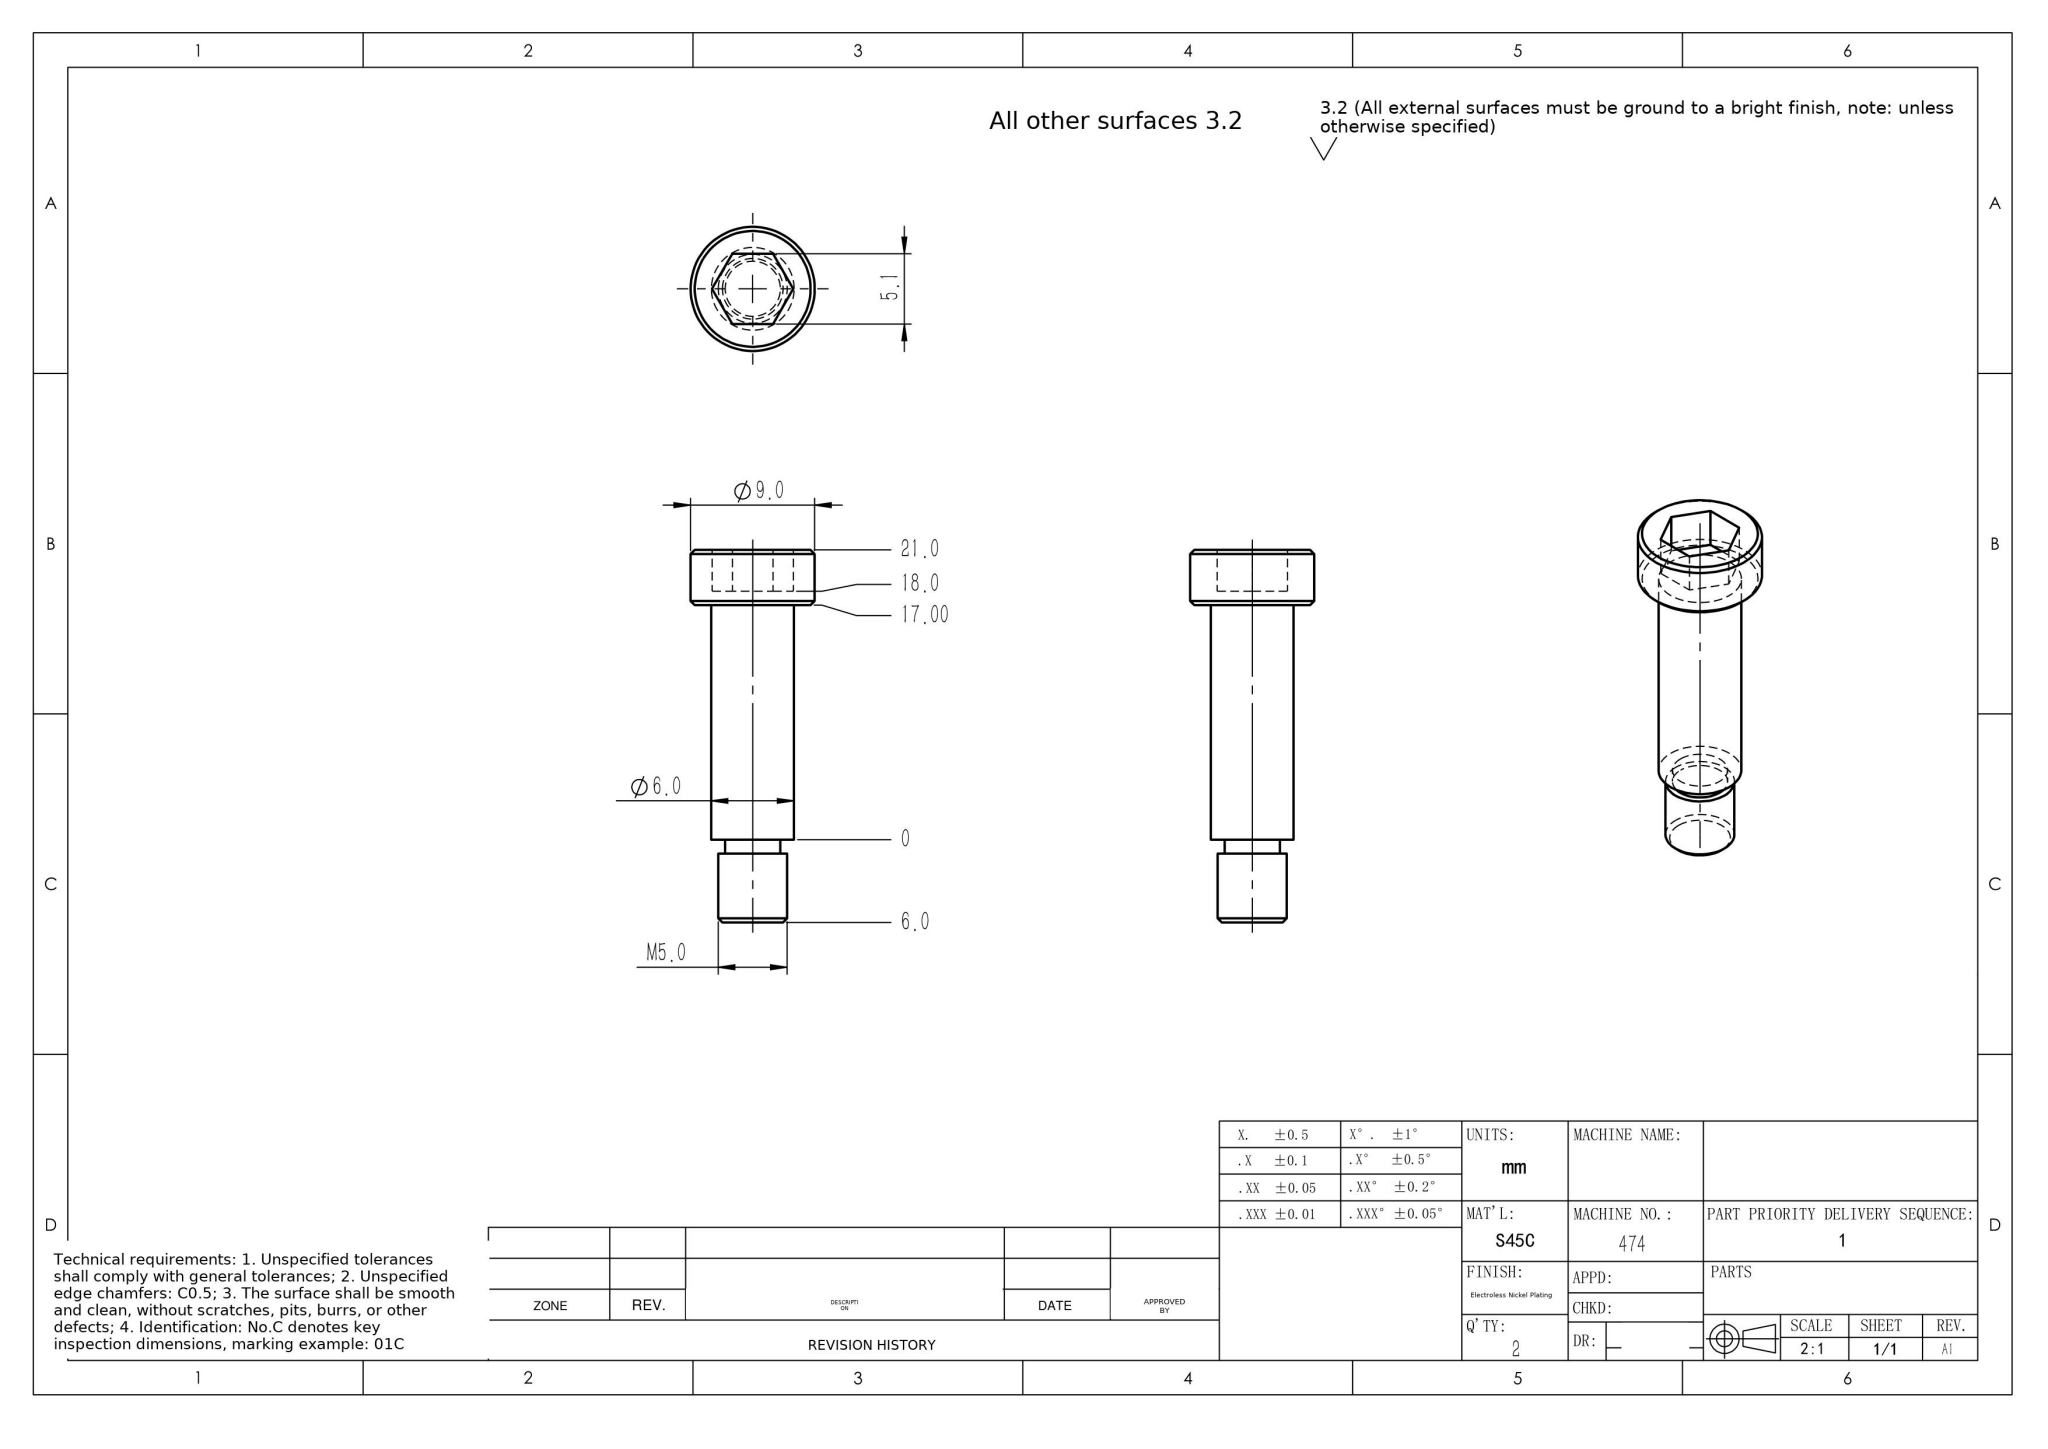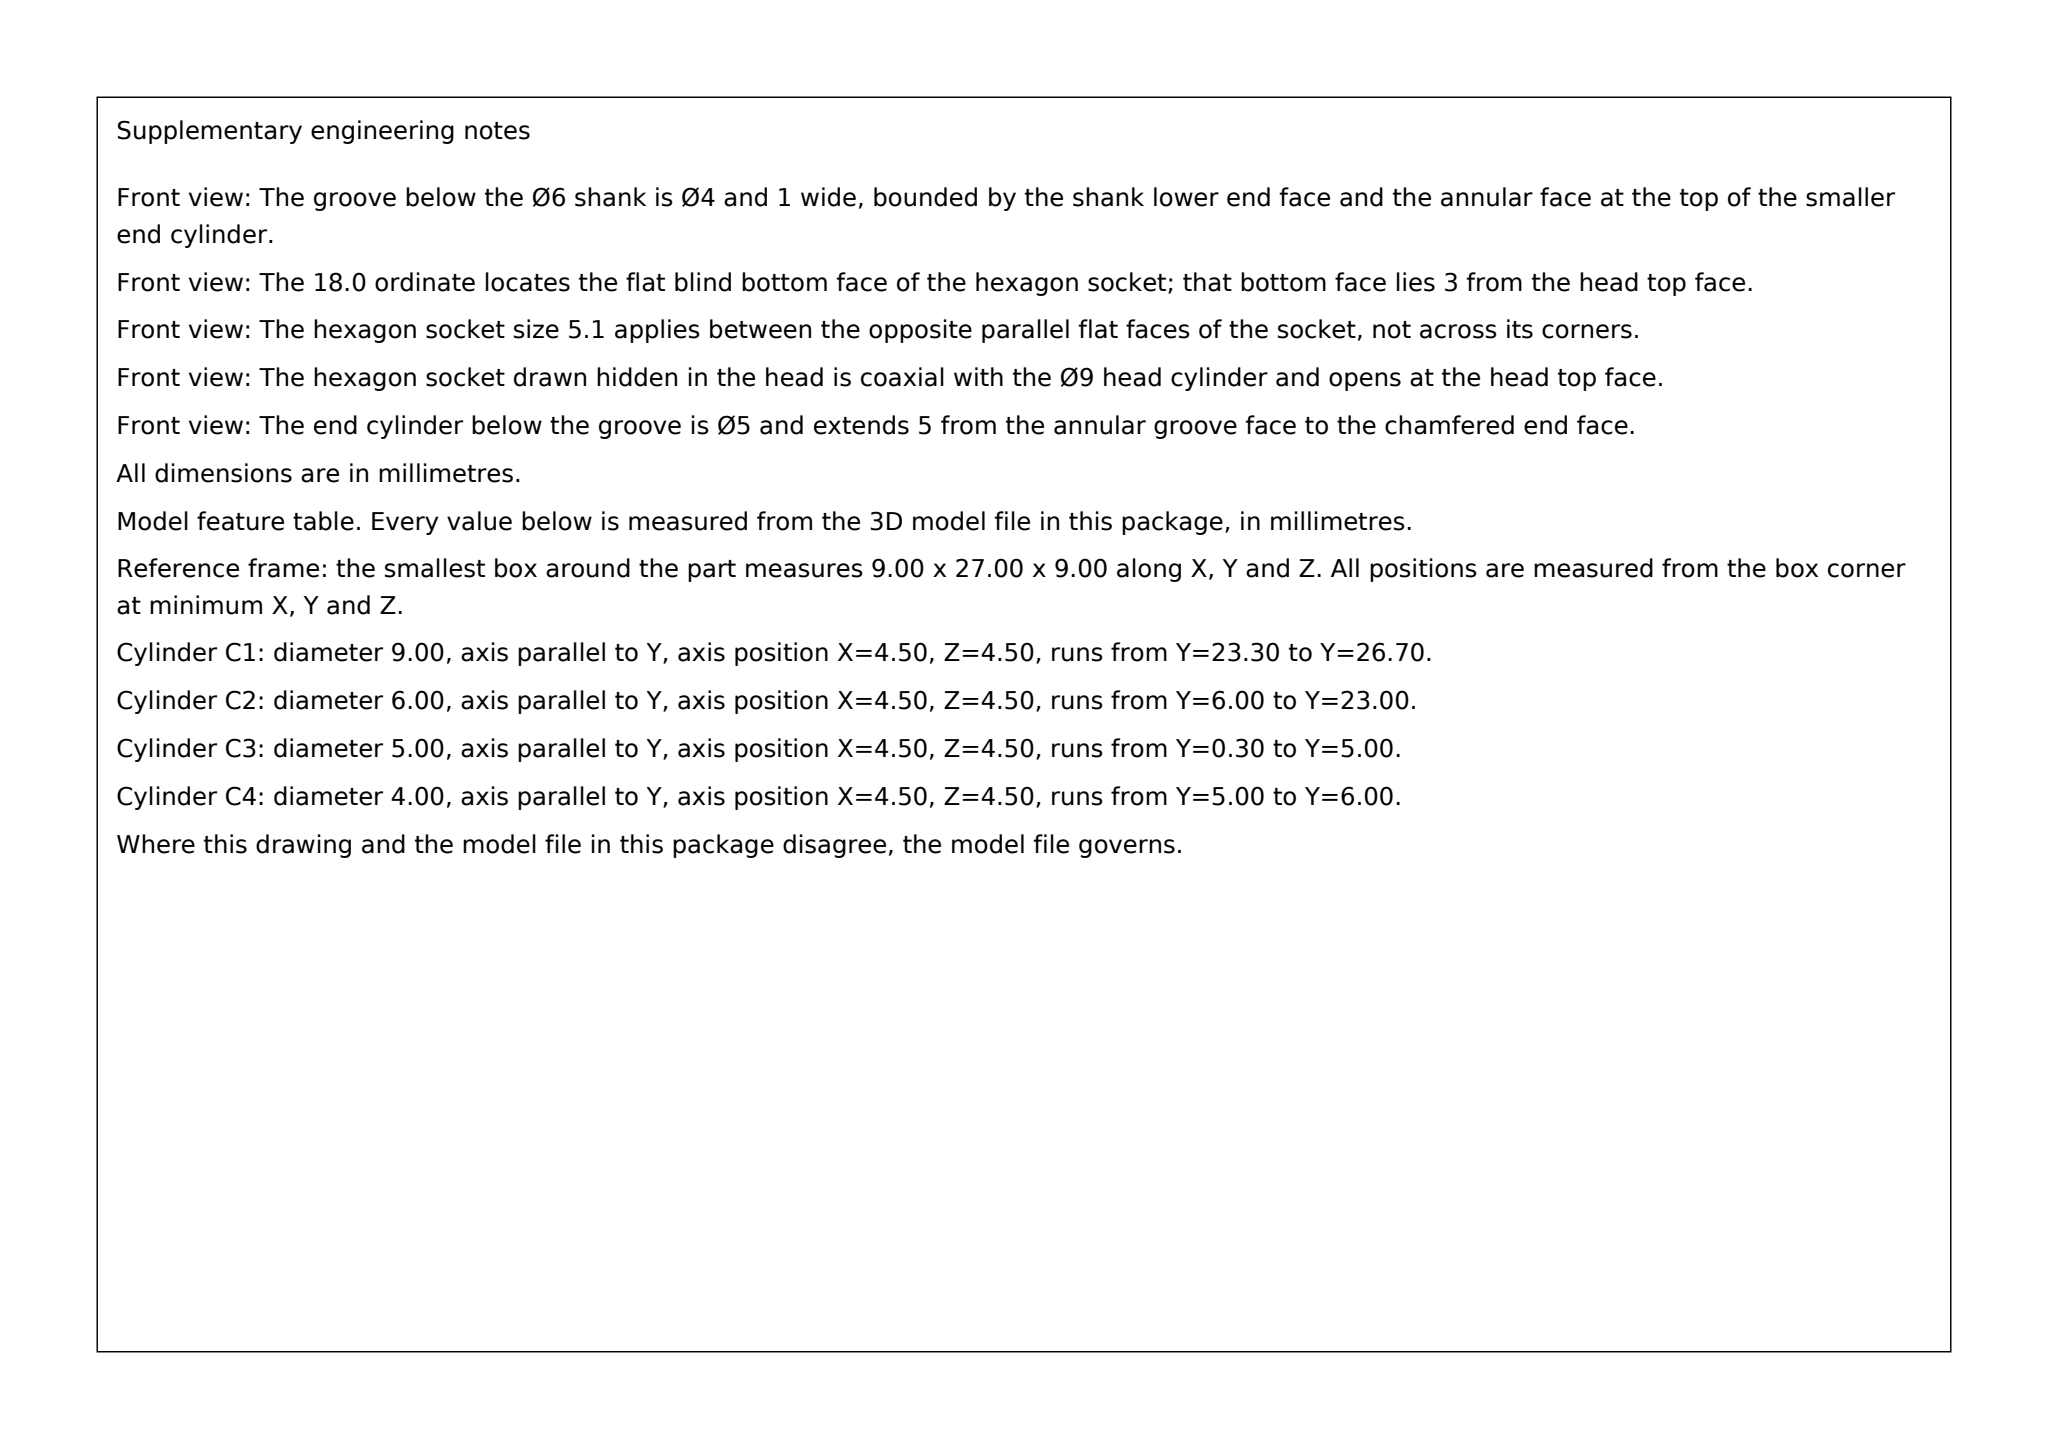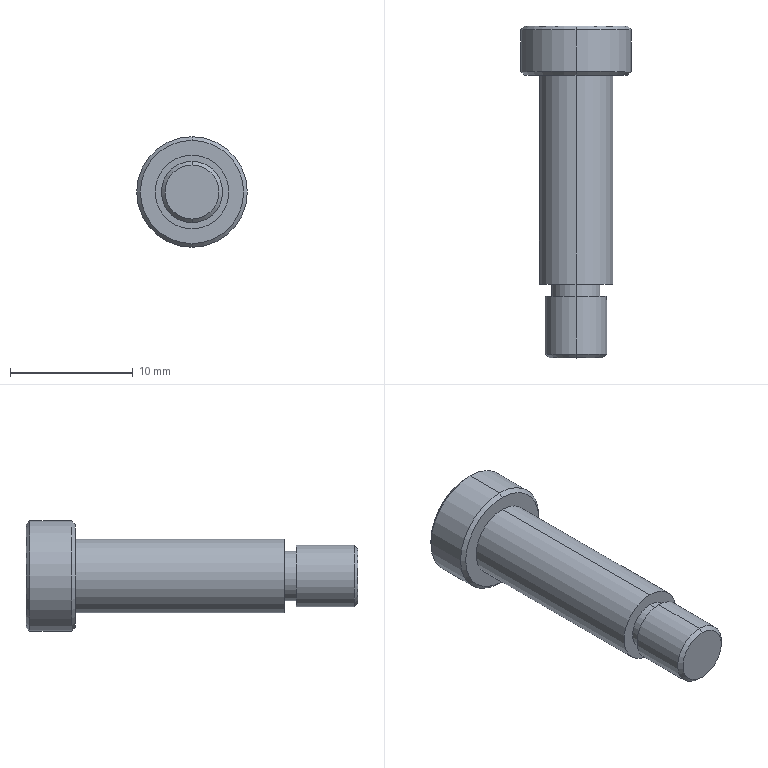Part | SolidWorks | mm | material S45C | 1 solid | 26 faces | box 9 x 27 x 9 mm | volume 775 mm3 | plane 12 | cylinder 8 | cone 6 | commonest cylinder face diameters 5 x2 4 x2 9 x2 6 x2
build123d program:
from build123d import *

# Parameters (mm, degrees)
SKETCH1_R           = 3
BOSS_EXTRUDE1_DEPTH = 17
SKETCH2_R           = 2.5
BOSS_EXTRUDE2_DEPTH = 6
SKETCH3_R           = 4.5
BOSS_EXTRUDE3_DEPTH = 4
CHAMFER1_SIZE       = 0.3
SKETCH4_W           = 1
SKETCH4_H           = 1
CUT_EXTRUDE1_DEPTH  = 3


with BuildPart() as part:
    # Sketch1 → Boss-Extrude1 (new body)
    with BuildSketch(Plane(origin=(0, 0, 0), x_dir=(1, 0, 0), z_dir=(0, 1, 0))):
        with Locations(Location((0, 0, 0), (0, 0, 270))):
            Circle(SKETCH1_R)
    extrude(amount=BOSS_EXTRUDE1_DEPTH)

    # Sketch2 → Boss-Extrude2 (add)
    with BuildSketch(Plane.XZ):
        with Locations(Location((0, 0, 0), (0, 0, 90))):
            Circle(SKETCH2_R)
    extrude(amount=BOSS_EXTRUDE2_DEPTH)

    # Sketch3 → Boss-Extrude3 (add)
    with BuildSketch(Plane(origin=(0, 17, 0), x_dir=(1, 0, 0), z_dir=(0, 1, 0))):
        with Locations(Location((0, 0, 0), (0, 0, 270))):
            Circle(SKETCH3_R)
    extrude(amount=BOSS_EXTRUDE3_DEPTH)

    # Chamfer1
    chamfer1_edges = [part.edges().sort_by_distance(p)[0] for p in [
        (0, -6, -2.5),
        (0, 17, -4.5),
        (0, 21, -4.5),
    ]]
    chamfer(chamfer1_edges, length=CHAMFER1_SIZE)

    # Sketch4 → Cut-Revolve1 (revolve, cut)
    with BuildSketch(Plane.XY, mode=Mode.PRIVATE) as cut_revolve1_sk:
        with Locations((2.5, -0.5)):
            Rectangle(SKETCH4_W, SKETCH4_H)
    revolve(cut_revolve1_sk.sketch.rotate(Axis((0, -5.7, 0), (0, 1, 0)), 90), axis=Axis((0, -5.7, 0), (0, 1, 0)), mode=Mode.SUBTRACT)

    # Sketch5 → Cut-Extrude1 (cut)
    with BuildSketch(Plane(origin=(0, 21, 0), x_dir=(1, 0, 0), z_dir=(0, 1, 0))):
        Polygon((0, 2.944), (-2.55, 1.472), (-2.55, -1.472), (0, -2.944), (2.55, -1.472), (2.55, 1.472), align=None)
    extrude(amount=-CUT_EXTRUDE1_DEPTH, mode=Mode.SUBTRACT)


solid = part.part
STEP:
#1=CARTESIAN_POINT('',(0.,-5.7,2.5));
#2=VERTEX_POINT('',#1);
#3=CARTESIAN_POINT('',(0.,-5.7,-2.5));
#4=VERTEX_POINT('',#3);
#5=CARTESIAN_POINT('',(0.,-5.7,0.));
#6=DIRECTION('',(0.,1.,0.));
#7=DIRECTION('',(0.,0.,-1.));
#8=AXIS2_PLACEMENT_3D('',#5,#6,#7);
#9=CIRCLE('',#8,2.5);
#10=EDGE_CURVE('',#2,#4,#9,.T.);
#11=ORIENTED_EDGE('',*,*,#10,.T.);
#12=CARTESIAN_POINT('',(0.,-1.,-2.5));
#13=VERTEX_POINT('',#12);
#14=CARTESIAN_POINT('',(0.,-6.,-2.5));
#15=DIRECTION('',(0.,1.,0.));
#16=VECTOR('',#15,1000.);
#17=LINE('',#14,#16);
#18=EDGE_CURVE('',#4,#13,#17,.T.);
#19=ORIENTED_EDGE('',*,*,#18,.T.);
#20=CARTESIAN_POINT('',(0.,-1.,2.5));
#21=VERTEX_POINT('',#20);
#22=CARTESIAN_POINT('',(0.,-1.,0.));
#23=DIRECTION('',(0.,-1.,0.));
#24=DIRECTION('',(0.,0.,-1.));
#25=AXIS2_PLACEMENT_3D('',#22,#23,#24);
#26=CIRCLE('',#25,2.5);
#27=EDGE_CURVE('',#13,#21,#26,.T.);
#28=ORIENTED_EDGE('',*,*,#27,.T.);
#29=CARTESIAN_POINT('',(0.,-6.,2.5));
#30=DIRECTION('',(0.,1.,0.));
#31=VECTOR('',#30,1000.);
#32=LINE('',#29,#31);
#33=EDGE_CURVE('',#2,#21,#32,.T.);
#34=ORIENTED_EDGE('',*,*,#33,.F.);
#35=EDGE_LOOP('',(#11,#19,#28,#34));
#36=FACE_OUTER_BOUND('',#35,.T.);
#37=CARTESIAN_POINT('',(0.,-6.,0.));
#38=DIRECTION('',(0.,1.,0.));
#39=DIRECTION('',(0.,0.,1.));
#40=AXIS2_PLACEMENT_3D('',#37,#38,#39);
#41=CYLINDRICAL_SURFACE('',#40,2.5);
#42=ADVANCED_FACE('',(#36),#41,.T.);
#43=CARTESIAN_POINT('',(0.,-6.,-2.2));
#44=VERTEX_POINT('',#43);
#45=CARTESIAN_POINT('',(0.,-6.,2.2));
#46=VERTEX_POINT('',#45);
#47=CARTESIAN_POINT('',(0.,-6.,0.));
#48=DIRECTION('',(0.,-1.,0.));
#49=DIRECTION('',(0.,0.,-1.));
#50=AXIS2_PLACEMENT_3D('',#47,#48,#49);
#51=CIRCLE('',#50,2.2);
#52=EDGE_CURVE('',#44,#46,#51,.T.);
#53=ORIENTED_EDGE('',*,*,#52,.F.);
#54=CARTESIAN_POINT('',(0.,-6.,-2.2));
#55=DIRECTION('',(0.,0.7071,-0.7071));
#56=VECTOR('',#55,1000.);
#57=LINE('',#54,#56);
#58=EDGE_CURVE('',#44,#4,#57,.T.);
#59=ORIENTED_EDGE('',*,*,#58,.T.);
#60=ORIENTED_EDGE('',*,*,#10,.F.);
#61=CARTESIAN_POINT('',(0.,-6.,2.2));
#62=DIRECTION('',(0.,0.7071,0.7071));
#63=VECTOR('',#62,1000.);
#64=LINE('',#61,#63);
#65=EDGE_CURVE('',#46,#2,#64,.T.);
#66=ORIENTED_EDGE('',*,*,#65,.F.);
#67=EDGE_LOOP('',(#53,#59,#60,#66));
#68=FACE_OUTER_BOUND('',#67,.T.);
#69=CARTESIAN_POINT('',(0.,-6.,0.));
#70=DIRECTION('',(0.,1.,0.));
#71=DIRECTION('',(0.,0.,1.));
#72=AXIS2_PLACEMENT_3D('',#69,#70,#71);
#73=CONICAL_SURFACE('',#72,2.2,0.7854);
#74=ADVANCED_FACE('',(#68),#73,.T.);
#75=CARTESIAN_POINT('',(0.,0.,-2.));
#76=VERTEX_POINT('',#75);
#77=CARTESIAN_POINT('',(0.,0.,2.));
#78=VERTEX_POINT('',#77);
#79=CARTESIAN_POINT('',(0.,0.,0.));
#80=DIRECTION('',(0.,-1.,0.));
#81=DIRECTION('',(0.,0.,-1.));
#82=AXIS2_PLACEMENT_3D('',#79,#80,#81);
#83=CIRCLE('',#82,2.);
#84=EDGE_CURVE('',#76,#78,#83,.T.);
#85=ORIENTED_EDGE('',*,*,#84,.T.);
#86=CARTESIAN_POINT('',(0.,-1.,2.));
#87=VERTEX_POINT('',#86);
#88=CARTESIAN_POINT('',(0.,-5.7,2.));
#89=DIRECTION('',(0.,-1.,0.));
#90=VECTOR('',#89,1000.);
#91=LINE('',#88,#90);
#92=EDGE_CURVE('',#78,#87,#91,.T.);
#93=ORIENTED_EDGE('',*,*,#92,.T.);
#94=CARTESIAN_POINT('',(0.,-1.,-2.));
#95=VERTEX_POINT('',#94);
#96=CARTESIAN_POINT('',(0.,-1.,0.));
#97=DIRECTION('',(0.,-1.,0.));
#98=DIRECTION('',(0.,0.,-1.));
#99=AXIS2_PLACEMENT_3D('',#96,#97,#98);
#100=CIRCLE('',#99,2.);
#101=EDGE_CURVE('',#95,#87,#100,.T.);
#102=ORIENTED_EDGE('',*,*,#101,.F.);
#103=CARTESIAN_POINT('',(0.,-5.7,-2.));
#104=DIRECTION('',(0.,-1.,0.));
#105=VECTOR('',#104,1000.);
#106=LINE('',#103,#105);
#107=EDGE_CURVE('',#76,#95,#106,.T.);
#108=ORIENTED_EDGE('',*,*,#107,.F.);
#109=EDGE_LOOP('',(#85,#93,#102,#108));
#110=FACE_OUTER_BOUND('',#109,.T.);
#111=CARTESIAN_POINT('',(0.,-5.7,0.));
#112=DIRECTION('',(0.,-1.,0.));
#113=DIRECTION('',(0.,0.,-1.));
#114=AXIS2_PLACEMENT_3D('',#111,#112,#113);
#115=CYLINDRICAL_SURFACE('',#114,2.);
#116=ADVANCED_FACE('',(#110),#115,.T.);
#117=CARTESIAN_POINT('',(0.,17.,-4.2));
#118=VERTEX_POINT('',#117);
#119=CARTESIAN_POINT('',(0.,17.,4.2));
#120=VERTEX_POINT('',#119);
#121=CARTESIAN_POINT('',(0.,17.,0.));
#122=DIRECTION('',(0.,-1.,0.));
#123=DIRECTION('',(0.,0.,1.));
#124=AXIS2_PLACEMENT_3D('',#121,#122,#123);
#125=CIRCLE('',#124,4.2);
#126=EDGE_CURVE('',#118,#120,#125,.T.);
#127=ORIENTED_EDGE('',*,*,#126,.F.);
#128=CARTESIAN_POINT('',(0.,17.3,-4.5));
#129=VERTEX_POINT('',#128);
#130=CARTESIAN_POINT('',(0.,17.3,-4.5));
#131=DIRECTION('',(0.,0.7071,-0.7071));
#132=VECTOR('',#131,1000.);
#133=LINE('',#130,#132);
#134=EDGE_CURVE('',#118,#129,#133,.T.);
#135=ORIENTED_EDGE('',*,*,#134,.T.);
#136=CARTESIAN_POINT('',(0.,17.3,4.5));
#137=VERTEX_POINT('',#136);
#138=CARTESIAN_POINT('',(0.,17.3,0.));
#139=DIRECTION('',(0.,1.,0.));
#140=DIRECTION('',(0.,0.,1.));
#141=AXIS2_PLACEMENT_3D('',#138,#139,#140);
#142=CIRCLE('',#141,4.5);
#143=EDGE_CURVE('',#137,#129,#142,.T.);
#144=ORIENTED_EDGE('',*,*,#143,.F.);
#145=CARTESIAN_POINT('',(0.,17.3,4.5));
#146=DIRECTION('',(0.,0.7071,0.7071));
#147=VECTOR('',#146,1000.);
#148=LINE('',#145,#147);
#149=EDGE_CURVE('',#120,#137,#148,.T.);
#150=ORIENTED_EDGE('',*,*,#149,.F.);
#151=EDGE_LOOP('',(#127,#135,#144,#150));
#152=FACE_OUTER_BOUND('',#151,.T.);
#153=CARTESIAN_POINT('',(0.,17.3,0.));
#154=DIRECTION('',(0.,1.,0.));
#155=DIRECTION('',(0.,0.,1.));
#156=AXIS2_PLACEMENT_3D('',#153,#154,#155);
#157=CONICAL_SURFACE('',#156,4.5,0.7854);
#158=ADVANCED_FACE('',(#152),#157,.T.);
#159=CARTESIAN_POINT('',(0.,21.,4.2));
#160=VERTEX_POINT('',#159);
#161=CARTESIAN_POINT('',(0.,21.,-4.2));
#162=VERTEX_POINT('',#161);
#163=CARTESIAN_POINT('',(0.,21.,0.));
#164=DIRECTION('',(0.,1.,0.));
#165=DIRECTION('',(0.,0.,1.));
#166=AXIS2_PLACEMENT_3D('',#163,#164,#165);
#167=CIRCLE('',#166,4.2);
#168=EDGE_CURVE('',#160,#162,#167,.T.);
#169=ORIENTED_EDGE('',*,*,#168,.F.);
#170=CARTESIAN_POINT('',(0.,20.7,4.5));
#171=VERTEX_POINT('',#170);
#172=CARTESIAN_POINT('',(0.,21.,4.2));
#173=DIRECTION('',(0.,-0.7071,0.7071));
#174=VECTOR('',#173,1000.);
#175=LINE('',#172,#174);
#176=EDGE_CURVE('',#160,#171,#175,.T.);
#177=ORIENTED_EDGE('',*,*,#176,.T.);
#178=CARTESIAN_POINT('',(0.,20.7,-4.5));
#179=VERTEX_POINT('',#178);
#180=CARTESIAN_POINT('',(0.,20.7,0.));
#181=DIRECTION('',(0.,-1.,0.));
#182=DIRECTION('',(0.,0.,1.));
#183=AXIS2_PLACEMENT_3D('',#180,#181,#182);
#184=CIRCLE('',#183,4.5);
#185=EDGE_CURVE('',#179,#171,#184,.T.);
#186=ORIENTED_EDGE('',*,*,#185,.F.);
#187=CARTESIAN_POINT('',(0.,21.,-4.2));
#188=DIRECTION('',(0.,-0.7071,-0.7071));
#189=VECTOR('',#188,1000.);
#190=LINE('',#187,#189);
#191=EDGE_CURVE('',#162,#179,#190,.T.);
#192=ORIENTED_EDGE('',*,*,#191,.F.);
#193=EDGE_LOOP('',(#169,#177,#186,#192));
#194=FACE_OUTER_BOUND('',#193,.T.);
#195=CARTESIAN_POINT('',(0.,21.,0.));
#196=DIRECTION('',(0.,-1.,0.));
#197=DIRECTION('',(0.,0.,-1.));
#198=AXIS2_PLACEMENT_3D('',#195,#196,#197);
#199=CONICAL_SURFACE('',#198,4.2,0.7854);
#200=ADVANCED_FACE('',(#194),#199,.T.);
#201=ORIENTED_EDGE('',*,*,#185,.T.);
#202=CARTESIAN_POINT('',(0.,21.,4.5));
#203=DIRECTION('',(0.,-1.,0.));
#204=VECTOR('',#203,1000.);
#205=LINE('',#202,#204);
#206=EDGE_CURVE('',#171,#137,#205,.T.);
#207=ORIENTED_EDGE('',*,*,#206,.T.);
#208=ORIENTED_EDGE('',*,*,#143,.T.);
#209=CARTESIAN_POINT('',(0.,21.,-4.5));
#210=DIRECTION('',(0.,-1.,0.));
#211=VECTOR('',#210,1000.);
#212=LINE('',#209,#211);
#213=EDGE_CURVE('',#179,#129,#212,.T.);
#214=ORIENTED_EDGE('',*,*,#213,.F.);
#215=EDGE_LOOP('',(#201,#207,#208,#214));
#216=FACE_OUTER_BOUND('',#215,.T.);
#217=CARTESIAN_POINT('',(0.,21.,0.));
#218=DIRECTION('',(0.,-1.,0.));
#219=DIRECTION('',(0.,0.,-1.));
#220=AXIS2_PLACEMENT_3D('',#217,#218,#219);
#221=CYLINDRICAL_SURFACE('',#220,4.5);
#222=ADVANCED_FACE('',(#216),#221,.T.);
#223=CARTESIAN_POINT('',(0.,17.,3.));
#224=VERTEX_POINT('',#223);
#225=CARTESIAN_POINT('',(0.,17.,-3.));
#226=VERTEX_POINT('',#225);
#227=CARTESIAN_POINT('',(0.,17.,0.));
#228=DIRECTION('',(0.,1.,0.));
#229=DIRECTION('',(0.,0.,1.));
#230=AXIS2_PLACEMENT_3D('',#227,#228,#229);
#231=CIRCLE('',#230,3.);
#232=EDGE_CURVE('',#224,#226,#231,.T.);
#233=ORIENTED_EDGE('',*,*,#232,.F.);
#234=CARTESIAN_POINT('',(0.,0.,3.));
#235=VERTEX_POINT('',#234);
#236=CARTESIAN_POINT('',(0.,17.,3.));
#237=DIRECTION('',(0.,-1.,0.));
#238=VECTOR('',#237,1000.);
#239=LINE('',#236,#238);
#240=EDGE_CURVE('',#224,#235,#239,.T.);
#241=ORIENTED_EDGE('',*,*,#240,.T.);
#242=CARTESIAN_POINT('',(0.,0.,-3.));
#243=VERTEX_POINT('',#242);
#244=CARTESIAN_POINT('',(0.,0.,0.));
#245=DIRECTION('',(0.,1.,0.));
#246=DIRECTION('',(0.,0.,1.));
#247=AXIS2_PLACEMENT_3D('',#244,#245,#246);
#248=CIRCLE('',#247,3.);
#249=EDGE_CURVE('',#235,#243,#248,.T.);
#250=ORIENTED_EDGE('',*,*,#249,.T.);
#251=CARTESIAN_POINT('',(0.,17.,-3.));
#252=DIRECTION('',(0.,-1.,0.));
#253=VECTOR('',#252,1000.);
#254=LINE('',#251,#253);
#255=EDGE_CURVE('',#226,#243,#254,.T.);
#256=ORIENTED_EDGE('',*,*,#255,.F.);
#257=EDGE_LOOP('',(#233,#241,#250,#256));
#258=FACE_OUTER_BOUND('',#257,.T.);
#259=CARTESIAN_POINT('',(0.,17.,0.));
#260=DIRECTION('',(0.,-1.,0.));
#261=DIRECTION('',(0.,0.,-1.));
#262=AXIS2_PLACEMENT_3D('',#259,#260,#261);
#263=CYLINDRICAL_SURFACE('',#262,3.);
#264=ADVANCED_FACE('',(#258),#263,.T.);
#265=ORIENTED_EDGE('',*,*,#240,.F.);
#266=CARTESIAN_POINT('',(0.,17.,0.));
#267=DIRECTION('',(0.,1.,0.));
#268=DIRECTION('',(0.,0.,1.));
#269=AXIS2_PLACEMENT_3D('',#266,#267,#268);
#270=CIRCLE('',#269,3.);
#271=EDGE_CURVE('',#226,#224,#270,.T.);
#272=ORIENTED_EDGE('',*,*,#271,.F.);
#273=ORIENTED_EDGE('',*,*,#255,.T.);
#274=CARTESIAN_POINT('',(0.,0.,0.));
#275=DIRECTION('',(0.,1.,0.));
#276=DIRECTION('',(0.,0.,1.));
#277=AXIS2_PLACEMENT_3D('',#274,#275,#276);
#278=CIRCLE('',#277,3.);
#279=EDGE_CURVE('',#243,#235,#278,.T.);
#280=ORIENTED_EDGE('',*,*,#279,.T.);
#281=EDGE_LOOP('',(#265,#272,#273,#280));
#282=FACE_OUTER_BOUND('',#281,.T.);
#283=CARTESIAN_POINT('',(0.,17.,0.));
#284=DIRECTION('',(0.,-1.,0.));
#285=DIRECTION('',(0.,0.,-1.));
#286=AXIS2_PLACEMENT_3D('',#283,#284,#285);
#287=CYLINDRICAL_SURFACE('',#286,3.);
#288=ADVANCED_FACE('',(#282),#287,.T.);
#289=ORIENTED_EDGE('',*,*,#279,.F.);
#290=ORIENTED_EDGE('',*,*,#249,.F.);
#291=EDGE_LOOP('',(#289,#290));
#292=FACE_OUTER_BOUND('',#291,.T.);
#293=ORIENTED_EDGE('',*,*,#84,.F.);
#294=CARTESIAN_POINT('',(0.,0.,0.));
#295=DIRECTION('',(0.,-1.,0.));
#296=DIRECTION('',(0.,0.,-1.));
#297=AXIS2_PLACEMENT_3D('',#294,#295,#296);
#298=CIRCLE('',#297,2.);
#299=EDGE_CURVE('',#78,#76,#298,.T.);
#300=ORIENTED_EDGE('',*,*,#299,.F.);
#301=EDGE_LOOP('',(#293,#300));
#302=FACE_BOUND('',#301,.T.);
#303=CARTESIAN_POINT('',(0.,0.,0.));
#304=DIRECTION('',(0.,1.,0.));
#305=DIRECTION('',(0.,0.,1.));
#306=AXIS2_PLACEMENT_3D('',#303,#304,#305);
#307=PLANE('',#306);
#308=ADVANCED_FACE('',(#292,#302),#307,.F.);
#309=ORIENTED_EDGE('',*,*,#206,.F.);
#310=CARTESIAN_POINT('',(0.,20.7,0.));
#311=DIRECTION('',(0.,-1.,0.));
#312=DIRECTION('',(0.,0.,1.));
#313=AXIS2_PLACEMENT_3D('',#310,#311,#312);
#314=CIRCLE('',#313,4.5);
#315=EDGE_CURVE('',#171,#179,#314,.T.);
#316=ORIENTED_EDGE('',*,*,#315,.T.);
#317=ORIENTED_EDGE('',*,*,#213,.T.);
#318=CARTESIAN_POINT('',(0.,17.3,0.));
#319=DIRECTION('',(0.,1.,0.));
#320=DIRECTION('',(0.,0.,1.));
#321=AXIS2_PLACEMENT_3D('',#318,#319,#320);
#322=CIRCLE('',#321,4.5);
#323=EDGE_CURVE('',#129,#137,#322,.T.);
#324=ORIENTED_EDGE('',*,*,#323,.T.);
#325=EDGE_LOOP('',(#309,#316,#317,#324));
#326=FACE_OUTER_BOUND('',#325,.T.);
#327=CARTESIAN_POINT('',(0.,21.,0.));
#328=DIRECTION('',(0.,-1.,0.));
#329=DIRECTION('',(0.,0.,-1.));
#330=AXIS2_PLACEMENT_3D('',#327,#328,#329);
#331=CYLINDRICAL_SURFACE('',#330,4.5);
#332=ADVANCED_FACE('',(#326),#331,.T.);
#333=CARTESIAN_POINT('',(2.55,21.,-1.472));
#334=VERTEX_POINT('',#333);
#335=CARTESIAN_POINT('',(0.,21.,-2.944));
#336=VERTEX_POINT('',#335);
#337=CARTESIAN_POINT('',(2.55,21.,-1.472));
#338=DIRECTION('',(-0.866,0.,-0.5));
#339=VECTOR('',#338,1000.);
#340=LINE('',#337,#339);
#341=EDGE_CURVE('',#334,#336,#340,.T.);
#342=ORIENTED_EDGE('',*,*,#341,.F.);
#343=CARTESIAN_POINT('',(2.55,21.,1.472));
#344=VERTEX_POINT('',#343);
#345=CARTESIAN_POINT('',(2.55,21.,1.472));
#346=DIRECTION('',(0.,0.,-1.));
#347=VECTOR('',#346,1000.);
#348=LINE('',#345,#347);
#349=EDGE_CURVE('',#344,#334,#348,.T.);
#350=ORIENTED_EDGE('',*,*,#349,.F.);
#351=CARTESIAN_POINT('',(0.,21.,2.944));
#352=VERTEX_POINT('',#351);
#353=CARTESIAN_POINT('',(0.,21.,2.944));
#354=DIRECTION('',(0.866,0.,-0.5));
#355=VECTOR('',#354,1000.);
#356=LINE('',#353,#355);
#357=EDGE_CURVE('',#352,#344,#356,.T.);
#358=ORIENTED_EDGE('',*,*,#357,.F.);
#359=CARTESIAN_POINT('',(-2.55,21.,1.472));
#360=VERTEX_POINT('',#359);
#361=CARTESIAN_POINT('',(-2.55,21.,1.472));
#362=DIRECTION('',(0.866,0.,0.5));
#363=VECTOR('',#362,1000.);
#364=LINE('',#361,#363);
#365=EDGE_CURVE('',#360,#352,#364,.T.);
#366=ORIENTED_EDGE('',*,*,#365,.F.);
#367=CARTESIAN_POINT('',(-2.55,21.,-1.472));
#368=VERTEX_POINT('',#367);
#369=CARTESIAN_POINT('',(-2.55,21.,-1.472));
#370=DIRECTION('',(0.,0.,1.));
#371=VECTOR('',#370,1000.);
#372=LINE('',#369,#371);
#373=EDGE_CURVE('',#368,#360,#372,.T.);
#374=ORIENTED_EDGE('',*,*,#373,.F.);
#375=CARTESIAN_POINT('',(0.,21.,-2.944));
#376=DIRECTION('',(-0.866,0.,0.5));
#377=VECTOR('',#376,1000.);
#378=LINE('',#375,#377);
#379=EDGE_CURVE('',#336,#368,#378,.T.);
#380=ORIENTED_EDGE('',*,*,#379,.F.);
#381=EDGE_LOOP('',(#342,#350,#358,#366,#374,#380));
#382=FACE_BOUND('',#381,.T.);
#383=CARTESIAN_POINT('',(0.,21.,0.));
#384=DIRECTION('',(0.,1.,0.));
#385=DIRECTION('',(0.,0.,1.));
#386=AXIS2_PLACEMENT_3D('',#383,#384,#385);
#387=CIRCLE('',#386,4.2);
#388=EDGE_CURVE('',#162,#160,#387,.T.);
#389=ORIENTED_EDGE('',*,*,#388,.T.);
#390=ORIENTED_EDGE('',*,*,#168,.T.);
#391=EDGE_LOOP('',(#389,#390));
#392=FACE_OUTER_BOUND('',#391,.T.);
#393=CARTESIAN_POINT('',(0.,21.,0.));
#394=DIRECTION('',(0.,1.,0.));
#395=DIRECTION('',(0.,0.,1.));
#396=AXIS2_PLACEMENT_3D('',#393,#394,#395);
#397=PLANE('',#396);
#398=ADVANCED_FACE('',(#382,#392),#397,.T.);
#399=CARTESIAN_POINT('',(0.,17.,0.));
#400=DIRECTION('',(0.,-1.,0.));
#401=DIRECTION('',(0.,0.,1.));
#402=AXIS2_PLACEMENT_3D('',#399,#400,#401);
#403=CIRCLE('',#402,4.2);
#404=EDGE_CURVE('',#120,#118,#403,.T.);
#405=ORIENTED_EDGE('',*,*,#404,.T.);
#406=ORIENTED_EDGE('',*,*,#126,.T.);
#407=EDGE_LOOP('',(#405,#406));
#408=FACE_OUTER_BOUND('',#407,.T.);
#409=ORIENTED_EDGE('',*,*,#271,.T.);
#410=ORIENTED_EDGE('',*,*,#232,.T.);
#411=EDGE_LOOP('',(#409,#410));
#412=FACE_BOUND('',#411,.T.);
#413=CARTESIAN_POINT('',(0.,17.,0.));
#414=DIRECTION('',(0.,1.,0.));
#415=DIRECTION('',(0.,0.,1.));
#416=AXIS2_PLACEMENT_3D('',#413,#414,#415);
#417=PLANE('',#416);
#418=ADVANCED_FACE('',(#408,#412),#417,.F.);
#419=ORIENTED_EDGE('',*,*,#176,.F.);
#420=ORIENTED_EDGE('',*,*,#388,.F.);
#421=ORIENTED_EDGE('',*,*,#191,.T.);
#422=ORIENTED_EDGE('',*,*,#315,.F.);
#423=EDGE_LOOP('',(#419,#420,#421,#422));
#424=FACE_OUTER_BOUND('',#423,.T.);
#425=CARTESIAN_POINT('',(0.,21.,0.));
#426=DIRECTION('',(0.,-1.,0.));
#427=DIRECTION('',(0.,0.,-1.));
#428=AXIS2_PLACEMENT_3D('',#425,#426,#427);
#429=CONICAL_SURFACE('',#428,4.2,0.7854);
#430=ADVANCED_FACE('',(#424),#429,.T.);
#431=ORIENTED_EDGE('',*,*,#134,.F.);
#432=ORIENTED_EDGE('',*,*,#404,.F.);
#433=ORIENTED_EDGE('',*,*,#149,.T.);
#434=ORIENTED_EDGE('',*,*,#323,.F.);
#435=EDGE_LOOP('',(#431,#432,#433,#434));
#436=FACE_OUTER_BOUND('',#435,.T.);
#437=CARTESIAN_POINT('',(0.,17.3,0.));
#438=DIRECTION('',(0.,1.,0.));
#439=DIRECTION('',(0.,0.,1.));
#440=AXIS2_PLACEMENT_3D('',#437,#438,#439);
#441=CONICAL_SURFACE('',#440,4.5,0.7854);
#442=ADVANCED_FACE('',(#436),#441,.T.);
#443=ORIENTED_EDGE('',*,*,#101,.T.);
#444=CARTESIAN_POINT('',(0.,-1.,0.));
#445=DIRECTION('',(0.,-1.,0.));
#446=DIRECTION('',(0.,0.,-1.));
#447=AXIS2_PLACEMENT_3D('',#444,#445,#446);
#448=CIRCLE('',#447,2.);
#449=EDGE_CURVE('',#87,#95,#448,.T.);
#450=ORIENTED_EDGE('',*,*,#449,.T.);
#451=EDGE_LOOP('',(#443,#450));
#452=FACE_BOUND('',#451,.T.);
#453=CARTESIAN_POINT('',(0.,-1.,0.));
#454=DIRECTION('',(0.,-1.,0.));
#455=DIRECTION('',(0.,0.,-1.));
#456=AXIS2_PLACEMENT_3D('',#453,#454,#455);
#457=CIRCLE('',#456,2.5);
#458=EDGE_CURVE('',#21,#13,#457,.T.);
#459=ORIENTED_EDGE('',*,*,#458,.F.);
#460=ORIENTED_EDGE('',*,*,#27,.F.);
#461=EDGE_LOOP('',(#459,#460));
#462=FACE_OUTER_BOUND('',#461,.T.);
#463=CARTESIAN_POINT('',(2.,-1.,0.));
#464=DIRECTION('',(0.,-1.,0.));
#465=DIRECTION('',(0.,0.,-1.));
#466=AXIS2_PLACEMENT_3D('',#463,#464,#465);
#467=PLANE('',#466);
#468=ADVANCED_FACE('',(#452,#462),#467,.F.);
#469=ORIENTED_EDGE('',*,*,#92,.F.);
#470=ORIENTED_EDGE('',*,*,#299,.T.);
#471=ORIENTED_EDGE('',*,*,#107,.T.);
#472=ORIENTED_EDGE('',*,*,#449,.F.);
#473=EDGE_LOOP('',(#469,#470,#471,#472));
#474=FACE_OUTER_BOUND('',#473,.T.);
#475=CARTESIAN_POINT('',(0.,-5.7,0.));
#476=DIRECTION('',(0.,-1.,0.));
#477=DIRECTION('',(0.,0.,-1.));
#478=AXIS2_PLACEMENT_3D('',#475,#476,#477);
#479=CYLINDRICAL_SURFACE('',#478,2.);
#480=ADVANCED_FACE('',(#474),#479,.T.);
#481=CARTESIAN_POINT('',(0.,-6.,0.));
#482=DIRECTION('',(0.,-1.,0.));
#483=DIRECTION('',(0.,0.,-1.));
#484=AXIS2_PLACEMENT_3D('',#481,#482,#483);
#485=CIRCLE('',#484,2.2);
#486=EDGE_CURVE('',#46,#44,#485,.T.);
#487=ORIENTED_EDGE('',*,*,#486,.T.);
#488=ORIENTED_EDGE('',*,*,#52,.T.);
#489=EDGE_LOOP('',(#487,#488));
#490=FACE_OUTER_BOUND('',#489,.T.);
#491=CARTESIAN_POINT('',(0.,-6.,0.));
#492=DIRECTION('',(0.,-1.,0.));
#493=DIRECTION('',(0.,0.,-1.));
#494=AXIS2_PLACEMENT_3D('',#491,#492,#493);
#495=PLANE('',#494);
#496=ADVANCED_FACE('',(#490),#495,.T.);
#497=ORIENTED_EDGE('',*,*,#58,.F.);
#498=ORIENTED_EDGE('',*,*,#486,.F.);
#499=ORIENTED_EDGE('',*,*,#65,.T.);
#500=CARTESIAN_POINT('',(0.,-5.7,0.));
#501=DIRECTION('',(0.,1.,0.));
#502=DIRECTION('',(0.,0.,-1.));
#503=AXIS2_PLACEMENT_3D('',#500,#501,#502);
#504=CIRCLE('',#503,2.5);
#505=EDGE_CURVE('',#4,#2,#504,.T.);
#506=ORIENTED_EDGE('',*,*,#505,.F.);
#507=EDGE_LOOP('',(#497,#498,#499,#506));
#508=FACE_OUTER_BOUND('',#507,.T.);
#509=CARTESIAN_POINT('',(0.,-6.,0.));
#510=DIRECTION('',(0.,1.,0.));
#511=DIRECTION('',(0.,0.,1.));
#512=AXIS2_PLACEMENT_3D('',#509,#510,#511);
#513=CONICAL_SURFACE('',#512,2.2,0.7854);
#514=ADVANCED_FACE('',(#508),#513,.T.);
#515=ORIENTED_EDGE('',*,*,#18,.F.);
#516=ORIENTED_EDGE('',*,*,#505,.T.);
#517=ORIENTED_EDGE('',*,*,#33,.T.);
#518=ORIENTED_EDGE('',*,*,#458,.T.);
#519=EDGE_LOOP('',(#515,#516,#517,#518));
#520=FACE_OUTER_BOUND('',#519,.T.);
#521=CARTESIAN_POINT('',(0.,-6.,0.));
#522=DIRECTION('',(0.,1.,0.));
#523=DIRECTION('',(0.,0.,1.));
#524=AXIS2_PLACEMENT_3D('',#521,#522,#523);
#525=CYLINDRICAL_SURFACE('',#524,2.5);
#526=ADVANCED_FACE('',(#520),#525,.T.);
#527=ORIENTED_EDGE('',*,*,#341,.T.);
#528=CARTESIAN_POINT('',(0.,18.,-2.944));
#529=VERTEX_POINT('',#528);
#530=CARTESIAN_POINT('',(0.,18.,-2.944));
#531=DIRECTION('',(0.,1.,0.));
#532=VECTOR('',#531,1000.);
#533=LINE('',#530,#532);
#534=EDGE_CURVE('',#529,#336,#533,.T.);
#535=ORIENTED_EDGE('',*,*,#534,.F.);
#536=CARTESIAN_POINT('',(2.55,18.,-1.472));
#537=VERTEX_POINT('',#536);
#538=CARTESIAN_POINT('',(2.55,18.,-1.472));
#539=DIRECTION('',(-0.866,0.,-0.5));
#540=VECTOR('',#539,1000.);
#541=LINE('',#538,#540);
#542=EDGE_CURVE('',#537,#529,#541,.T.);
#543=ORIENTED_EDGE('',*,*,#542,.F.);
#544=CARTESIAN_POINT('',(2.55,18.,-1.472));
#545=DIRECTION('',(0.,1.,0.));
#546=VECTOR('',#545,1000.);
#547=LINE('',#544,#546);
#548=EDGE_CURVE('',#537,#334,#547,.T.);
#549=ORIENTED_EDGE('',*,*,#548,.T.);
#550=EDGE_LOOP('',(#527,#535,#543,#549));
#551=FACE_OUTER_BOUND('',#550,.T.);
#552=CARTESIAN_POINT('',(2.55,18.,-1.472));
#553=DIRECTION('',(0.5,0.,-0.866));
#554=DIRECTION('',(-0.866,0.,-0.5));
#555=AXIS2_PLACEMENT_3D('',#552,#553,#554);
#556=PLANE('',#555);
#557=ADVANCED_FACE('',(#551),#556,.F.);
#558=ORIENTED_EDGE('',*,*,#349,.T.);
#559=ORIENTED_EDGE('',*,*,#548,.F.);
#560=CARTESIAN_POINT('',(2.55,18.,1.472));
#561=VERTEX_POINT('',#560);
#562=CARTESIAN_POINT('',(2.55,18.,1.472));
#563=DIRECTION('',(0.,0.,-1.));
#564=VECTOR('',#563,1000.);
#565=LINE('',#562,#564);
#566=EDGE_CURVE('',#561,#537,#565,.T.);
#567=ORIENTED_EDGE('',*,*,#566,.F.);
#568=CARTESIAN_POINT('',(2.55,18.,1.472));
#569=DIRECTION('',(0.,1.,0.));
#570=VECTOR('',#569,1000.);
#571=LINE('',#568,#570);
#572=EDGE_CURVE('',#561,#344,#571,.T.);
#573=ORIENTED_EDGE('',*,*,#572,.T.);
#574=EDGE_LOOP('',(#558,#559,#567,#573));
#575=FACE_OUTER_BOUND('',#574,.T.);
#576=CARTESIAN_POINT('',(2.55,18.,1.472));
#577=DIRECTION('',(1.,0.,0.));
#578=DIRECTION('',(0.,0.,-1.));
#579=AXIS2_PLACEMENT_3D('',#576,#577,#578);
#580=PLANE('',#579);
#581=ADVANCED_FACE('',(#575),#580,.F.);
#582=ORIENTED_EDGE('',*,*,#357,.T.);
#583=ORIENTED_EDGE('',*,*,#572,.F.);
#584=CARTESIAN_POINT('',(0.,18.,2.944));
#585=VERTEX_POINT('',#584);
#586=CARTESIAN_POINT('',(0.,18.,2.944));
#587=DIRECTION('',(0.866,0.,-0.5));
#588=VECTOR('',#587,1000.);
#589=LINE('',#586,#588);
#590=EDGE_CURVE('',#585,#561,#589,.T.);
#591=ORIENTED_EDGE('',*,*,#590,.F.);
#592=CARTESIAN_POINT('',(0.,18.,2.944));
#593=DIRECTION('',(0.,1.,0.));
#594=VECTOR('',#593,1000.);
#595=LINE('',#592,#594);
#596=EDGE_CURVE('',#585,#352,#595,.T.);
#597=ORIENTED_EDGE('',*,*,#596,.T.);
#598=EDGE_LOOP('',(#582,#583,#591,#597));
#599=FACE_OUTER_BOUND('',#598,.T.);
#600=CARTESIAN_POINT('',(0.,18.,2.944));
#601=DIRECTION('',(0.5,0.,0.866));
#602=DIRECTION('',(0.866,0.,-0.5));
#603=AXIS2_PLACEMENT_3D('',#600,#601,#602);
#604=PLANE('',#603);
#605=ADVANCED_FACE('',(#599),#604,.F.);
#606=ORIENTED_EDGE('',*,*,#365,.T.);
#607=ORIENTED_EDGE('',*,*,#596,.F.);
#608=CARTESIAN_POINT('',(-2.55,18.,1.472));
#609=VERTEX_POINT('',#608);
#610=CARTESIAN_POINT('',(-2.55,18.,1.472));
#611=DIRECTION('',(0.866,0.,0.5));
#612=VECTOR('',#611,1000.);
#613=LINE('',#610,#612);
#614=EDGE_CURVE('',#609,#585,#613,.T.);
#615=ORIENTED_EDGE('',*,*,#614,.F.);
#616=CARTESIAN_POINT('',(-2.55,18.,1.472));
#617=DIRECTION('',(0.,1.,0.));
#618=VECTOR('',#617,1000.);
#619=LINE('',#616,#618);
#620=EDGE_CURVE('',#609,#360,#619,.T.);
#621=ORIENTED_EDGE('',*,*,#620,.T.);
#622=EDGE_LOOP('',(#606,#607,#615,#621));
#623=FACE_OUTER_BOUND('',#622,.T.);
#624=CARTESIAN_POINT('',(-2.55,18.,1.472));
#625=DIRECTION('',(-0.5,0.,0.866));
#626=DIRECTION('',(0.866,0.,0.5));
#627=AXIS2_PLACEMENT_3D('',#624,#625,#626);
#628=PLANE('',#627);
#629=ADVANCED_FACE('',(#623),#628,.F.);
#630=ORIENTED_EDGE('',*,*,#373,.T.);
#631=ORIENTED_EDGE('',*,*,#620,.F.);
#632=CARTESIAN_POINT('',(-2.55,18.,-1.472));
#633=VERTEX_POINT('',#632);
#634=CARTESIAN_POINT('',(-2.55,18.,-1.472));
#635=DIRECTION('',(0.,0.,1.));
#636=VECTOR('',#635,1000.);
#637=LINE('',#634,#636);
#638=EDGE_CURVE('',#633,#609,#637,.T.);
#639=ORIENTED_EDGE('',*,*,#638,.F.);
#640=CARTESIAN_POINT('',(-2.55,18.,-1.472));
#641=DIRECTION('',(0.,1.,0.));
#642=VECTOR('',#641,1000.);
#643=LINE('',#640,#642);
#644=EDGE_CURVE('',#633,#368,#643,.T.);
#645=ORIENTED_EDGE('',*,*,#644,.T.);
#646=EDGE_LOOP('',(#630,#631,#639,#645));
#647=FACE_OUTER_BOUND('',#646,.T.);
#648=CARTESIAN_POINT('',(-2.55,18.,-1.472));
#649=DIRECTION('',(-1.,0.,0.));
#650=DIRECTION('',(0.,0.,1.));
#651=AXIS2_PLACEMENT_3D('',#648,#649,#650);
#652=PLANE('',#651);
#653=ADVANCED_FACE('',(#647),#652,.F.);
#654=ORIENTED_EDGE('',*,*,#379,.T.);
#655=ORIENTED_EDGE('',*,*,#644,.F.);
#656=CARTESIAN_POINT('',(0.,18.,-2.944));
#657=DIRECTION('',(-0.866,0.,0.5));
#658=VECTOR('',#657,1000.);
#659=LINE('',#656,#658);
#660=EDGE_CURVE('',#529,#633,#659,.T.);
#661=ORIENTED_EDGE('',*,*,#660,.F.);
#662=ORIENTED_EDGE('',*,*,#534,.T.);
#663=EDGE_LOOP('',(#654,#655,#661,#662));
#664=FACE_OUTER_BOUND('',#663,.T.);
#665=CARTESIAN_POINT('',(0.,18.,-2.944));
#666=DIRECTION('',(-0.5,0.,-0.866));
#667=DIRECTION('',(-0.866,0.,0.5));
#668=AXIS2_PLACEMENT_3D('',#665,#666,#667);
#669=PLANE('',#668);
#670=ADVANCED_FACE('',(#664),#669,.F.);
#671=ORIENTED_EDGE('',*,*,#542,.T.);
#672=ORIENTED_EDGE('',*,*,#660,.T.);
#673=ORIENTED_EDGE('',*,*,#638,.T.);
#674=ORIENTED_EDGE('',*,*,#614,.T.);
#675=ORIENTED_EDGE('',*,*,#590,.T.);
#676=ORIENTED_EDGE('',*,*,#566,.T.);
#677=EDGE_LOOP('',(#671,#672,#673,#674,#675,#676));
#678=FACE_OUTER_BOUND('',#677,.T.);
#679=CARTESIAN_POINT('',(0.,18.,0.));
#680=DIRECTION('',(0.,1.,0.));
#681=DIRECTION('',(0.,0.,1.));
#682=AXIS2_PLACEMENT_3D('',#679,#680,#681);
#683=PLANE('',#682);
#684=ADVANCED_FACE('',(#678),#683,.T.);
#685=CLOSED_SHELL('',(#42,#74,#116,#158,#200,#222,#264,#288,#308,#332,#398,#418,#430,#442,#468,#480,#496,#514,#526,#557,#581,#605,#629,#653,#670,#684));
#686=MANIFOLD_SOLID_BREP('',#685);
#687=CARTESIAN_POINT('',(0.,0.,0.));
#688=DIRECTION('',(0.,0.,1.));
#689=DIRECTION('',(1.,0.,0.));
#690=AXIS2_PLACEMENT_3D('',#687,#688,#689);
#691=(LENGTH_UNIT()NAMED_UNIT(*)SI_UNIT(.MILLI.,.METRE.));
#692=UNCERTAINTY_MEASURE_WITH_UNIT(LENGTH_MEASURE(0.00001),#691,'','');
#693=(NAMED_UNIT(*)PLANE_ANGLE_UNIT()SI_UNIT($,.RADIAN.));
#694=(NAMED_UNIT(*)SI_UNIT($,.STERADIAN.)SOLID_ANGLE_UNIT());
#695=(GEOMETRIC_REPRESENTATION_CONTEXT(3)GLOBAL_UNCERTAINTY_ASSIGNED_CONTEXT((#692))GLOBAL_UNIT_ASSIGNED_CONTEXT((#691,#693,#694))REPRESENTATION_CONTEXT('',''));
#696=ADVANCED_BREP_SHAPE_REPRESENTATION('',(#686,#690),#695);